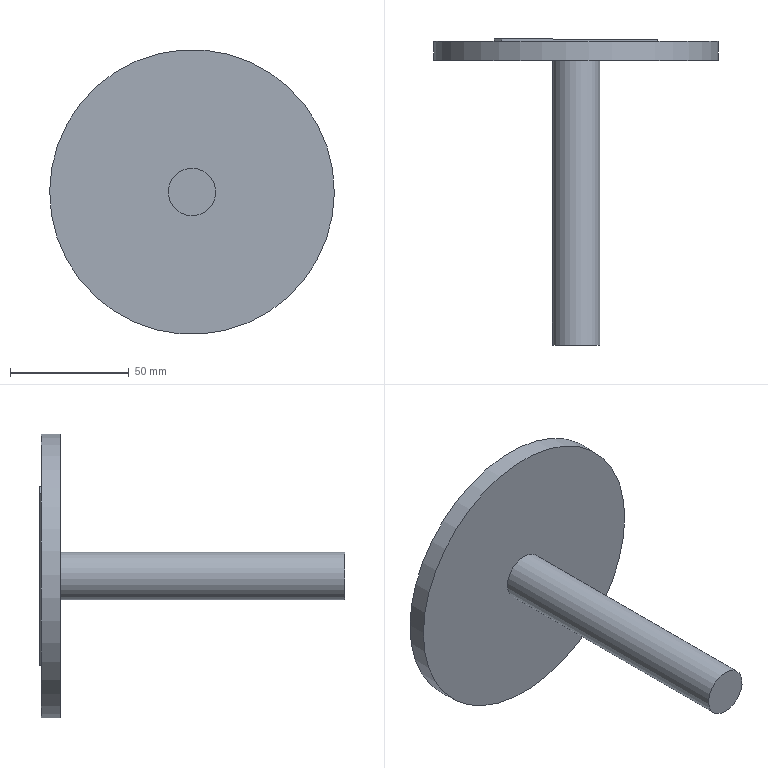Component | NX | MODEL3_3 | 1 solid | 10 faces | box 120 x 129 x 120 mm | volume 128614 mm3 | plane 8 | cylinder 2 | commonest cylinder face diameters 120 x1 20 x1
STEP:
#1=CARTESIAN_POINT('',(0.,0.,0.));
#2=DIRECTION('',(0.,0.,1.));
#3=DIRECTION('',(1.,0.,0.));
#4=AXIS2_PLACEMENT_3D('',#1,#2,#3);
#5=CARTESIAN_POINT('',(-22.229,260.,-82.788));
#6=VERTEX_POINT('',#5);
#7=CARTESIAN_POINT('',(-62.472,260.,-38.286));
#8=DIRECTION('',(0.,-1.,0.));
#9=DIRECTION('',(0.6707,0.,-0.7417));
#10=AXIS2_PLACEMENT_3D('',#7,#8,#9);
#11=CIRCLE('',#10,60.);
#12=CARTESIAN_POINT('',(-62.472,260.,-38.286));
#13=DIRECTION('',(0.,-1.,0.));
#14=DIRECTION('',(-0.7417,0.,-0.6707));
#15=AXIS2_PLACEMENT_3D('',#12,#13,#14);
#16=PLANE('',#15);
#17=CARTESIAN_POINT('',(0.,0.));
#18=DIRECTION('',(0.,1.));
#19=AXIS2_PLACEMENT_2D('',#17,#18);
#20=CIRCLE('',#19,60.);
#21=(GEOMETRIC_REPRESENTATION_CONTEXT(2)PARAMETRIC_REPRESENTATION_CONTEXT()REPRESENTATION_CONTEXT('',''));
#22=DEFINITIONAL_REPRESENTATION('',(#20),#21);
#23=PCURVE('',#16,#22);
#24=CARTESIAN_POINT('',(-62.472,252.,-38.286));
#25=DIRECTION('',(0.,1.,0.));
#26=DIRECTION('',(0.7417,0.,0.6707));
#27=AXIS2_PLACEMENT_3D('',#24,#25,#26);
#28=CYLINDRICAL_SURFACE('',#27,60.);
#29=CARTESIAN_POINT('',(7.854,8.));
#30=DIRECTION('',(-1.,0.));
#31=VECTOR('',#30,1.);
#32=LINE('',#29,#31);
#33=(GEOMETRIC_REPRESENTATION_CONTEXT(2)PARAMETRIC_REPRESENTATION_CONTEXT()REPRESENTATION_CONTEXT('',''));
#34=DEFINITIONAL_REPRESENTATION('',(#32),#33);
#35=PCURVE('',#28,#34);
#36=SURFACE_CURVE('',#11,(#23,#35),.PCURVE_S1.);
#37=EDGE_CURVE('',#6,#6,#36,.T.);
#38=ORIENTED_EDGE('',*,*,#37,.F.);
#39=EDGE_LOOP('',(#38));
#40=FACE_BOUND('',#39,.T.);
#41=CARTESIAN_POINT('',(-96.993,260.,-3.439));
#42=VERTEX_POINT('',#41);
#43=CARTESIAN_POINT('',(-93.683,260.,-0.4456));
#44=VERTEX_POINT('',#43);
#45=CARTESIAN_POINT('',(-96.993,260.,-3.439));
#46=DIRECTION('',(0.7417,0.,0.6707));
#47=VECTOR('',#46,1.);
#48=LINE('',#45,#47);
#49=CARTESIAN_POINT('',(2.231,-49.));
#50=DIRECTION('',(-1.,0.));
#51=VECTOR('',#50,1.);
#52=LINE('',#49,#51);
#53=(GEOMETRIC_REPRESENTATION_CONTEXT(2)PARAMETRIC_REPRESENTATION_CONTEXT()REPRESENTATION_CONTEXT('',''));
#54=DEFINITIONAL_REPRESENTATION('',(#52),#53);
#55=PCURVE('',#16,#54);
#56=CARTESIAN_POINT('',(-96.993,261.,-3.439));
#57=DIRECTION('',(0.6707,0.,-0.7417));
#58=DIRECTION('',(0.7417,0.,0.6707));
#59=AXIS2_PLACEMENT_3D('',#56,#57,#58);
#60=PLANE('',#59);
#61=CARTESIAN_POINT('',(0.,1.));
#62=DIRECTION('',(1.,0.));
#63=VECTOR('',#62,1.);
#64=LINE('',#61,#63);
#65=(GEOMETRIC_REPRESENTATION_CONTEXT(2)PARAMETRIC_REPRESENTATION_CONTEXT()REPRESENTATION_CONTEXT('',''));
#66=DEFINITIONAL_REPRESENTATION('',(#64),#65);
#67=PCURVE('',#60,#66);
#68=SURFACE_CURVE('',#48,(#55,#67),.PCURVE_S1.);
#69=EDGE_CURVE('',#42,#44,#68,.T.);
#70=ORIENTED_EDGE('',*,*,#69,.F.);
#71=CARTESIAN_POINT('',(-31.262,260.,-76.126));
#72=VERTEX_POINT('',#71);
#73=CARTESIAN_POINT('',(-31.262,260.,-76.126));
#74=DIRECTION('',(-0.6707,0.,0.7417));
#75=VECTOR('',#74,1.);
#76=LINE('',#73,#75);
#77=CARTESIAN_POINT('',(2.231,49.));
#78=DIRECTION('',(0.,-1.));
#79=VECTOR('',#78,1.);
#80=LINE('',#77,#79);
#81=(GEOMETRIC_REPRESENTATION_CONTEXT(2)PARAMETRIC_REPRESENTATION_CONTEXT()REPRESENTATION_CONTEXT('',''));
#82=DEFINITIONAL_REPRESENTATION('',(#80),#81);
#83=PCURVE('',#16,#82);
#84=CARTESIAN_POINT('',(-31.262,261.,-76.126));
#85=DIRECTION('',(0.7417,0.,0.6707));
#86=DIRECTION('',(0.,-1.,0.));
#87=AXIS2_PLACEMENT_3D('',#84,#85,#86);
#88=PLANE('',#87);
#89=CARTESIAN_POINT('',(1.,0.));
#90=DIRECTION('',(0.,-1.));
#91=VECTOR('',#90,1.);
#92=LINE('',#89,#91);
#93=(GEOMETRIC_REPRESENTATION_CONTEXT(2)PARAMETRIC_REPRESENTATION_CONTEXT()REPRESENTATION_CONTEXT('',''));
#94=DEFINITIONAL_REPRESENTATION('',(#92),#93);
#95=PCURVE('',#88,#94);
#96=SURFACE_CURVE('',#76,(#83,#95),.PCURVE_S1.);
#97=EDGE_CURVE('',#72,#42,#96,.T.);
#98=ORIENTED_EDGE('',*,*,#97,.F.);
#99=CARTESIAN_POINT('',(-27.952,260.,-73.133));
#100=VERTEX_POINT('',#99);
#101=CARTESIAN_POINT('',(-27.952,260.,-73.133));
#102=DIRECTION('',(-0.7417,0.,-0.6707));
#103=VECTOR('',#102,1.);
#104=LINE('',#101,#103);
#105=CARTESIAN_POINT('',(-2.231,49.));
#106=DIRECTION('',(1.,-0.));
#107=VECTOR('',#106,1.);
#108=LINE('',#105,#107);
#109=(GEOMETRIC_REPRESENTATION_CONTEXT(2)PARAMETRIC_REPRESENTATION_CONTEXT()REPRESENTATION_CONTEXT('',''));
#110=DEFINITIONAL_REPRESENTATION('',(#108),#109);
#111=PCURVE('',#16,#110);
#112=CARTESIAN_POINT('',(-27.952,261.,-73.133));
#113=DIRECTION('',(-0.6707,0.,0.7417));
#114=DIRECTION('',(-0.7417,0.,-0.6707));
#115=AXIS2_PLACEMENT_3D('',#112,#113,#114);
#116=PLANE('',#115);
#117=CARTESIAN_POINT('',(0.,1.));
#118=DIRECTION('',(1.,0.));
#119=VECTOR('',#118,1.);
#120=LINE('',#117,#119);
#121=(GEOMETRIC_REPRESENTATION_CONTEXT(2)PARAMETRIC_REPRESENTATION_CONTEXT()REPRESENTATION_CONTEXT('',''));
#122=DEFINITIONAL_REPRESENTATION('',(#120),#121);
#123=PCURVE('',#116,#122);
#124=SURFACE_CURVE('',#104,(#111,#123),.PCURVE_S1.);
#125=EDGE_CURVE('',#100,#72,#124,.T.);
#126=ORIENTED_EDGE('',*,*,#125,.F.);
#127=CARTESIAN_POINT('',(-93.683,260.,-0.4456));
#128=DIRECTION('',(0.6707,0.,-0.7417));
#129=VECTOR('',#128,1.);
#130=LINE('',#127,#129);
#131=CARTESIAN_POINT('',(-2.231,-49.));
#132=DIRECTION('',(0.,1.));
#133=VECTOR('',#132,1.);
#134=LINE('',#131,#133);
#135=(GEOMETRIC_REPRESENTATION_CONTEXT(2)PARAMETRIC_REPRESENTATION_CONTEXT()REPRESENTATION_CONTEXT('',''));
#136=DEFINITIONAL_REPRESENTATION('',(#134),#135);
#137=PCURVE('',#16,#136);
#138=CARTESIAN_POINT('',(-93.683,261.,-0.4456));
#139=DIRECTION('',(-0.7417,0.,-0.6707));
#140=DIRECTION('',(0.,1.,0.));
#141=AXIS2_PLACEMENT_3D('',#138,#139,#140);
#142=PLANE('',#141);
#143=CARTESIAN_POINT('',(-1.,0.));
#144=DIRECTION('',(0.,1.));
#145=VECTOR('',#144,1.);
#146=LINE('',#143,#145);
#147=(GEOMETRIC_REPRESENTATION_CONTEXT(2)PARAMETRIC_REPRESENTATION_CONTEXT()REPRESENTATION_CONTEXT('',''));
#148=DEFINITIONAL_REPRESENTATION('',(#146),#147);
#149=PCURVE('',#142,#148);
#150=SURFACE_CURVE('',#130,(#137,#149),.PCURVE_S1.);
#151=EDGE_CURVE('',#44,#100,#150,.T.);
#152=ORIENTED_EDGE('',*,*,#151,.F.);
#153=EDGE_LOOP('',(#70,#98,#126,#152));
#154=FACE_BOUND('',#153,.T.);
#155=ADVANCED_FACE('',(#40,#154),#16,.F.);
#156=CARTESIAN_POINT('',(-22.229,252.,-82.788));
#157=VERTEX_POINT('',#156);
#158=CARTESIAN_POINT('',(-62.472,252.,-38.286));
#159=DIRECTION('',(0.,-1.,0.));
#160=DIRECTION('',(0.6707,0.,-0.7417));
#161=AXIS2_PLACEMENT_3D('',#158,#159,#160);
#162=CIRCLE('',#161,60.);
#163=CARTESIAN_POINT('',(7.854,0.));
#164=DIRECTION('',(-1.,0.));
#165=VECTOR('',#164,1.);
#166=LINE('',#163,#165);
#167=(GEOMETRIC_REPRESENTATION_CONTEXT(2)PARAMETRIC_REPRESENTATION_CONTEXT()REPRESENTATION_CONTEXT('',''));
#168=DEFINITIONAL_REPRESENTATION('',(#166),#167);
#169=PCURVE('',#28,#168);
#170=CARTESIAN_POINT('',(-62.472,252.,-38.286));
#171=DIRECTION('',(0.,-1.,0.));
#172=DIRECTION('',(-0.7417,0.,-0.6707));
#173=AXIS2_PLACEMENT_3D('',#170,#171,#172);
#174=PLANE('',#173);
#175=CARTESIAN_POINT('',(0.,0.));
#176=DIRECTION('',(0.,1.));
#177=AXIS2_PLACEMENT_2D('',#175,#176);
#178=CIRCLE('',#177,60.);
#179=(GEOMETRIC_REPRESENTATION_CONTEXT(2)PARAMETRIC_REPRESENTATION_CONTEXT()REPRESENTATION_CONTEXT('',''));
#180=DEFINITIONAL_REPRESENTATION('',(#178),#179);
#181=PCURVE('',#174,#180);
#182=SURFACE_CURVE('',#162,(#169,#181),.PCURVE_S1.);
#183=EDGE_CURVE('',#157,#157,#182,.T.);
#184=ORIENTED_EDGE('',*,*,#183,.F.);
#185=CARTESIAN_POINT('',(-22.229,252.,-82.788));
#186=CARTESIAN_POINT('',(-22.229,260.,-82.788));
#187=B_SPLINE_CURVE_WITH_KNOTS('',1,(#185,#186),.UNSPECIFIED.,.F.,.F.,(2,2),(0.,8.),.PIECEWISE_BEZIER_KNOTS.);
#188=CARTESIAN_POINT('',(7.854,0.));
#189=DIRECTION('',(0.,1.));
#190=VECTOR('',#189,1.);
#191=LINE('',#188,#190);
#192=(GEOMETRIC_REPRESENTATION_CONTEXT(2)PARAMETRIC_REPRESENTATION_CONTEXT()REPRESENTATION_CONTEXT('',''));
#193=DEFINITIONAL_REPRESENTATION('',(#191),#192);
#194=PCURVE('',#28,#193);
#195=CARTESIAN_POINT('',(1.571,0.));
#196=DIRECTION('',(0.,1.));
#197=VECTOR('',#196,1.);
#198=LINE('',#195,#197);
#199=(GEOMETRIC_REPRESENTATION_CONTEXT(2)PARAMETRIC_REPRESENTATION_CONTEXT()REPRESENTATION_CONTEXT('',''));
#200=DEFINITIONAL_REPRESENTATION('',(#198),#199);
#201=PCURVE('',#28,#200);
#202=SEAM_CURVE('',#187,(#194,#201),.PCURVE_S1.);
#203=EDGE_CURVE('',#157,#6,#202,.T.);
#204=ORIENTED_EDGE('',*,*,#203,.T.);
#205=ORIENTED_EDGE('',*,*,#37,.T.);
#206=ORIENTED_EDGE('',*,*,#203,.F.);
#207=EDGE_LOOP('',(#184,#204,#205,#206));
#208=FACE_BOUND('',#207,.T.);
#209=ADVANCED_FACE('',(#208),#28,.T.);
#210=CARTESIAN_POINT('',(-55.765,252.,-45.703));
#211=VERTEX_POINT('',#210);
#212=CARTESIAN_POINT('',(-62.472,252.,-38.286));
#213=DIRECTION('',(0.,-1.,0.));
#214=DIRECTION('',(0.6707,0.,-0.7417));
#215=AXIS2_PLACEMENT_3D('',#212,#213,#214);
#216=CIRCLE('',#215,10.);
#217=CARTESIAN_POINT('',(0.,0.));
#218=DIRECTION('',(-0.,1.));
#219=AXIS2_PLACEMENT_2D('',#217,#218);
#220=CIRCLE('',#219,10.);
#221=(GEOMETRIC_REPRESENTATION_CONTEXT(2)PARAMETRIC_REPRESENTATION_CONTEXT()REPRESENTATION_CONTEXT('',''));
#222=DEFINITIONAL_REPRESENTATION('',(#220),#221);
#223=PCURVE('',#174,#222);
#224=CARTESIAN_POINT('',(-62.472,132.,-38.286));
#225=DIRECTION('',(0.,1.,0.));
#226=DIRECTION('',(0.7417,0.,0.6707));
#227=AXIS2_PLACEMENT_3D('',#224,#225,#226);
#228=CYLINDRICAL_SURFACE('',#227,10.);
#229=CARTESIAN_POINT('',(7.854,120.));
#230=DIRECTION('',(-1.,0.));
#231=VECTOR('',#230,1.);
#232=LINE('',#229,#231);
#233=(GEOMETRIC_REPRESENTATION_CONTEXT(2)PARAMETRIC_REPRESENTATION_CONTEXT()REPRESENTATION_CONTEXT('',''));
#234=DEFINITIONAL_REPRESENTATION('',(#232),#233);
#235=PCURVE('',#228,#234);
#236=SURFACE_CURVE('',#216,(#223,#235),.PCURVE_S1.);
#237=EDGE_CURVE('',#211,#211,#236,.T.);
#238=ORIENTED_EDGE('',*,*,#237,.F.);
#239=EDGE_LOOP('',(#238));
#240=FACE_BOUND('',#239,.T.);
#241=ORIENTED_EDGE('',*,*,#183,.T.);
#242=EDGE_LOOP('',(#241));
#243=FACE_BOUND('',#242,.T.);
#244=ADVANCED_FACE('',(#240,#243),#174,.T.);
#245=CARTESIAN_POINT('',(-55.765,132.,-45.703));
#246=VERTEX_POINT('',#245);
#247=CARTESIAN_POINT('',(-62.472,132.,-38.286));
#248=DIRECTION('',(0.,-1.,0.));
#249=DIRECTION('',(0.6707,0.,-0.7417));
#250=AXIS2_PLACEMENT_3D('',#247,#248,#249);
#251=CIRCLE('',#250,10.);
#252=CARTESIAN_POINT('',(7.854,0.));
#253=DIRECTION('',(-1.,0.));
#254=VECTOR('',#253,1.);
#255=LINE('',#252,#254);
#256=(GEOMETRIC_REPRESENTATION_CONTEXT(2)PARAMETRIC_REPRESENTATION_CONTEXT()REPRESENTATION_CONTEXT('',''));
#257=DEFINITIONAL_REPRESENTATION('',(#255),#256);
#258=PCURVE('',#228,#257);
#259=CARTESIAN_POINT('',(-62.472,132.,-38.286));
#260=DIRECTION('',(0.,-1.,0.));
#261=DIRECTION('',(-0.7417,0.,-0.6707));
#262=AXIS2_PLACEMENT_3D('',#259,#260,#261);
#263=PLANE('',#262);
#264=CARTESIAN_POINT('',(0.,0.));
#265=DIRECTION('',(-0.,1.));
#266=AXIS2_PLACEMENT_2D('',#264,#265);
#267=CIRCLE('',#266,10.);
#268=(GEOMETRIC_REPRESENTATION_CONTEXT(2)PARAMETRIC_REPRESENTATION_CONTEXT()REPRESENTATION_CONTEXT('',''));
#269=DEFINITIONAL_REPRESENTATION('',(#267),#268);
#270=PCURVE('',#263,#269);
#271=SURFACE_CURVE('',#251,(#258,#270),.PCURVE_S1.);
#272=EDGE_CURVE('',#246,#246,#271,.T.);
#273=ORIENTED_EDGE('',*,*,#272,.F.);
#274=CARTESIAN_POINT('',(-55.765,132.,-45.703));
#275=CARTESIAN_POINT('',(-55.765,252.,-45.703));
#276=B_SPLINE_CURVE_WITH_KNOTS('',1,(#274,#275),.UNSPECIFIED.,.F.,.F.,(2,2),(0.,120.),.PIECEWISE_BEZIER_KNOTS.);
#277=CARTESIAN_POINT('',(7.854,0.));
#278=DIRECTION('',(0.,1.));
#279=VECTOR('',#278,1.);
#280=LINE('',#277,#279);
#281=(GEOMETRIC_REPRESENTATION_CONTEXT(2)PARAMETRIC_REPRESENTATION_CONTEXT()REPRESENTATION_CONTEXT('',''));
#282=DEFINITIONAL_REPRESENTATION('',(#280),#281);
#283=PCURVE('',#228,#282);
#284=CARTESIAN_POINT('',(1.571,0.));
#285=DIRECTION('',(0.,1.));
#286=VECTOR('',#285,1.);
#287=LINE('',#284,#286);
#288=(GEOMETRIC_REPRESENTATION_CONTEXT(2)PARAMETRIC_REPRESENTATION_CONTEXT()REPRESENTATION_CONTEXT('',''));
#289=DEFINITIONAL_REPRESENTATION('',(#287),#288);
#290=PCURVE('',#228,#289);
#291=SEAM_CURVE('',#276,(#283,#290),.PCURVE_S1.);
#292=EDGE_CURVE('',#246,#211,#291,.T.);
#293=ORIENTED_EDGE('',*,*,#292,.T.);
#294=ORIENTED_EDGE('',*,*,#237,.T.);
#295=ORIENTED_EDGE('',*,*,#292,.F.);
#296=EDGE_LOOP('',(#273,#293,#294,#295));
#297=FACE_BOUND('',#296,.T.);
#298=ADVANCED_FACE('',(#297),#228,.T.);
#299=ORIENTED_EDGE('',*,*,#272,.T.);
#300=EDGE_LOOP('',(#299));
#301=FACE_BOUND('',#300,.T.);
#302=ADVANCED_FACE('',(#301),#263,.T.);
#303=ORIENTED_EDGE('',*,*,#69,.T.);
#304=CARTESIAN_POINT('',(-93.683,261.,-0.4456));
#305=VERTEX_POINT('',#304);
#306=CARTESIAN_POINT('',(-93.683,261.,-0.4456));
#307=DIRECTION('',(0.,-1.,0.));
#308=VECTOR('',#307,1.);
#309=LINE('',#306,#308);
#310=CARTESIAN_POINT('',(4.462,0.));
#311=DIRECTION('',(0.,1.));
#312=VECTOR('',#311,1.);
#313=LINE('',#310,#312);
#314=(GEOMETRIC_REPRESENTATION_CONTEXT(2)PARAMETRIC_REPRESENTATION_CONTEXT()REPRESENTATION_CONTEXT('',''));
#315=DEFINITIONAL_REPRESENTATION('',(#313),#314);
#316=PCURVE('',#60,#315);
#317=CARTESIAN_POINT('',(0.,0.));
#318=DIRECTION('',(-1.,0.));
#319=VECTOR('',#318,1.);
#320=LINE('',#317,#319);
#321=(GEOMETRIC_REPRESENTATION_CONTEXT(2)PARAMETRIC_REPRESENTATION_CONTEXT()REPRESENTATION_CONTEXT('',''));
#322=DEFINITIONAL_REPRESENTATION('',(#320),#321);
#323=PCURVE('',#142,#322);
#324=SURFACE_CURVE('',#309,(#316,#323),.PCURVE_S1.);
#325=EDGE_CURVE('',#305,#44,#324,.T.);
#326=ORIENTED_EDGE('',*,*,#325,.F.);
#327=CARTESIAN_POINT('',(-96.993,261.,-3.439));
#328=VERTEX_POINT('',#327);
#329=CARTESIAN_POINT('',(-96.993,261.,-3.439));
#330=DIRECTION('',(0.7417,0.,0.6707));
#331=VECTOR('',#330,1.);
#332=LINE('',#329,#331);
#333=CARTESIAN_POINT('',(0.,0.));
#334=DIRECTION('',(1.,0.));
#335=VECTOR('',#334,1.);
#336=LINE('',#333,#335);
#337=(GEOMETRIC_REPRESENTATION_CONTEXT(2)PARAMETRIC_REPRESENTATION_CONTEXT()REPRESENTATION_CONTEXT('',''));
#338=DEFINITIONAL_REPRESENTATION('',(#336),#337);
#339=PCURVE('',#60,#338);
#340=CARTESIAN_POINT('',(-62.472,261.,-38.286));
#341=DIRECTION('',(0.,1.,0.));
#342=DIRECTION('',(0.7417,0.,0.6707));
#343=AXIS2_PLACEMENT_3D('',#340,#341,#342);
#344=PLANE('',#343);
#345=CARTESIAN_POINT('',(-2.231,-49.));
#346=DIRECTION('',(1.,0.));
#347=VECTOR('',#346,1.);
#348=LINE('',#345,#347);
#349=(GEOMETRIC_REPRESENTATION_CONTEXT(2)PARAMETRIC_REPRESENTATION_CONTEXT()REPRESENTATION_CONTEXT('',''));
#350=DEFINITIONAL_REPRESENTATION('',(#348),#349);
#351=PCURVE('',#344,#350);
#352=SURFACE_CURVE('',#332,(#339,#351),.PCURVE_S1.);
#353=EDGE_CURVE('',#328,#305,#352,.T.);
#354=ORIENTED_EDGE('',*,*,#353,.F.);
#355=CARTESIAN_POINT('',(-96.993,261.,-3.439));
#356=DIRECTION('',(0.,-1.,0.));
#357=VECTOR('',#356,1.);
#358=LINE('',#355,#357);
#359=CARTESIAN_POINT('',(0.,0.));
#360=DIRECTION('',(0.,1.));
#361=VECTOR('',#360,1.);
#362=LINE('',#359,#361);
#363=(GEOMETRIC_REPRESENTATION_CONTEXT(2)PARAMETRIC_REPRESENTATION_CONTEXT()REPRESENTATION_CONTEXT('',''));
#364=DEFINITIONAL_REPRESENTATION('',(#362),#363);
#365=PCURVE('',#60,#364);
#366=CARTESIAN_POINT('',(0.,-98.));
#367=DIRECTION('',(1.,0.));
#368=VECTOR('',#367,1.);
#369=LINE('',#366,#368);
#370=(GEOMETRIC_REPRESENTATION_CONTEXT(2)PARAMETRIC_REPRESENTATION_CONTEXT()REPRESENTATION_CONTEXT('',''));
#371=DEFINITIONAL_REPRESENTATION('',(#369),#370);
#372=PCURVE('',#88,#371);
#373=SURFACE_CURVE('',#358,(#365,#372),.PCURVE_S1.);
#374=EDGE_CURVE('',#328,#42,#373,.T.);
#375=ORIENTED_EDGE('',*,*,#374,.T.);
#376=EDGE_LOOP('',(#303,#326,#354,#375));
#377=FACE_BOUND('',#376,.T.);
#378=ADVANCED_FACE('',(#377),#60,.F.);
#379=ORIENTED_EDGE('',*,*,#151,.T.);
#380=CARTESIAN_POINT('',(-27.952,261.,-73.133));
#381=VERTEX_POINT('',#380);
#382=CARTESIAN_POINT('',(-27.952,261.,-73.133));
#383=DIRECTION('',(0.,-1.,0.));
#384=VECTOR('',#383,1.);
#385=LINE('',#382,#384);
#386=CARTESIAN_POINT('',(0.,98.));
#387=DIRECTION('',(-1.,0.));
#388=VECTOR('',#387,1.);
#389=LINE('',#386,#388);
#390=(GEOMETRIC_REPRESENTATION_CONTEXT(2)PARAMETRIC_REPRESENTATION_CONTEXT()REPRESENTATION_CONTEXT('',''));
#391=DEFINITIONAL_REPRESENTATION('',(#389),#390);
#392=PCURVE('',#142,#391);
#393=CARTESIAN_POINT('',(0.,0.));
#394=DIRECTION('',(0.,1.));
#395=VECTOR('',#394,1.);
#396=LINE('',#393,#395);
#397=(GEOMETRIC_REPRESENTATION_CONTEXT(2)PARAMETRIC_REPRESENTATION_CONTEXT()REPRESENTATION_CONTEXT('',''));
#398=DEFINITIONAL_REPRESENTATION('',(#396),#397);
#399=PCURVE('',#116,#398);
#400=SURFACE_CURVE('',#385,(#392,#399),.PCURVE_S1.);
#401=EDGE_CURVE('',#381,#100,#400,.T.);
#402=ORIENTED_EDGE('',*,*,#401,.F.);
#403=CARTESIAN_POINT('',(-93.683,261.,-0.4456));
#404=DIRECTION('',(0.6707,0.,-0.7417));
#405=VECTOR('',#404,1.);
#406=LINE('',#403,#405);
#407=CARTESIAN_POINT('',(0.,0.));
#408=DIRECTION('',(0.,1.));
#409=VECTOR('',#408,1.);
#410=LINE('',#407,#409);
#411=(GEOMETRIC_REPRESENTATION_CONTEXT(2)PARAMETRIC_REPRESENTATION_CONTEXT()REPRESENTATION_CONTEXT('',''));
#412=DEFINITIONAL_REPRESENTATION('',(#410),#411);
#413=PCURVE('',#142,#412);
#414=CARTESIAN_POINT('',(2.231,-49.));
#415=DIRECTION('',(0.,1.));
#416=VECTOR('',#415,1.);
#417=LINE('',#414,#416);
#418=(GEOMETRIC_REPRESENTATION_CONTEXT(2)PARAMETRIC_REPRESENTATION_CONTEXT()REPRESENTATION_CONTEXT('',''));
#419=DEFINITIONAL_REPRESENTATION('',(#417),#418);
#420=PCURVE('',#344,#419);
#421=SURFACE_CURVE('',#406,(#413,#420),.PCURVE_S1.);
#422=EDGE_CURVE('',#305,#381,#421,.T.);
#423=ORIENTED_EDGE('',*,*,#422,.F.);
#424=ORIENTED_EDGE('',*,*,#325,.T.);
#425=EDGE_LOOP('',(#379,#402,#423,#424));
#426=FACE_BOUND('',#425,.T.);
#427=ADVANCED_FACE('',(#426),#142,.F.);
#428=ORIENTED_EDGE('',*,*,#125,.T.);
#429=CARTESIAN_POINT('',(-31.262,261.,-76.126));
#430=VERTEX_POINT('',#429);
#431=CARTESIAN_POINT('',(-31.262,261.,-76.126));
#432=DIRECTION('',(0.,-1.,0.));
#433=VECTOR('',#432,1.);
#434=LINE('',#431,#433);
#435=CARTESIAN_POINT('',(4.462,0.));
#436=DIRECTION('',(0.,1.));
#437=VECTOR('',#436,1.);
#438=LINE('',#435,#437);
#439=(GEOMETRIC_REPRESENTATION_CONTEXT(2)PARAMETRIC_REPRESENTATION_CONTEXT()REPRESENTATION_CONTEXT('',''));
#440=DEFINITIONAL_REPRESENTATION('',(#438),#439);
#441=PCURVE('',#116,#440);
#442=CARTESIAN_POINT('',(0.,0.));
#443=DIRECTION('',(1.,0.));
#444=VECTOR('',#443,1.);
#445=LINE('',#442,#444);
#446=(GEOMETRIC_REPRESENTATION_CONTEXT(2)PARAMETRIC_REPRESENTATION_CONTEXT()REPRESENTATION_CONTEXT('',''));
#447=DEFINITIONAL_REPRESENTATION('',(#445),#446);
#448=PCURVE('',#88,#447);
#449=SURFACE_CURVE('',#434,(#441,#448),.PCURVE_S1.);
#450=EDGE_CURVE('',#430,#72,#449,.T.);
#451=ORIENTED_EDGE('',*,*,#450,.F.);
#452=CARTESIAN_POINT('',(-27.952,261.,-73.133));
#453=DIRECTION('',(-0.7417,0.,-0.6707));
#454=VECTOR('',#453,1.);
#455=LINE('',#452,#454);
#456=CARTESIAN_POINT('',(0.,0.));
#457=DIRECTION('',(1.,0.));
#458=VECTOR('',#457,1.);
#459=LINE('',#456,#458);
#460=(GEOMETRIC_REPRESENTATION_CONTEXT(2)PARAMETRIC_REPRESENTATION_CONTEXT()REPRESENTATION_CONTEXT('',''));
#461=DEFINITIONAL_REPRESENTATION('',(#459),#460);
#462=PCURVE('',#116,#461);
#463=CARTESIAN_POINT('',(2.231,49.));
#464=DIRECTION('',(-1.,-0.));
#465=VECTOR('',#464,1.);
#466=LINE('',#463,#465);
#467=(GEOMETRIC_REPRESENTATION_CONTEXT(2)PARAMETRIC_REPRESENTATION_CONTEXT()REPRESENTATION_CONTEXT('',''));
#468=DEFINITIONAL_REPRESENTATION('',(#466),#467);
#469=PCURVE('',#344,#468);
#470=SURFACE_CURVE('',#455,(#462,#469),.PCURVE_S1.);
#471=EDGE_CURVE('',#381,#430,#470,.T.);
#472=ORIENTED_EDGE('',*,*,#471,.F.);
#473=ORIENTED_EDGE('',*,*,#401,.T.);
#474=EDGE_LOOP('',(#428,#451,#472,#473));
#475=FACE_BOUND('',#474,.T.);
#476=ADVANCED_FACE('',(#475),#116,.F.);
#477=ORIENTED_EDGE('',*,*,#97,.T.);
#478=ORIENTED_EDGE('',*,*,#374,.F.);
#479=CARTESIAN_POINT('',(-31.262,261.,-76.126));
#480=DIRECTION('',(-0.6707,0.,0.7417));
#481=VECTOR('',#480,1.);
#482=LINE('',#479,#481);
#483=CARTESIAN_POINT('',(0.,0.));
#484=DIRECTION('',(0.,-1.));
#485=VECTOR('',#484,1.);
#486=LINE('',#483,#485);
#487=(GEOMETRIC_REPRESENTATION_CONTEXT(2)PARAMETRIC_REPRESENTATION_CONTEXT()REPRESENTATION_CONTEXT('',''));
#488=DEFINITIONAL_REPRESENTATION('',(#486),#487);
#489=PCURVE('',#88,#488);
#490=CARTESIAN_POINT('',(-2.231,49.));
#491=DIRECTION('',(0.,-1.));
#492=VECTOR('',#491,1.);
#493=LINE('',#490,#492);
#494=(GEOMETRIC_REPRESENTATION_CONTEXT(2)PARAMETRIC_REPRESENTATION_CONTEXT()REPRESENTATION_CONTEXT('',''));
#495=DEFINITIONAL_REPRESENTATION('',(#493),#494);
#496=PCURVE('',#344,#495);
#497=SURFACE_CURVE('',#482,(#489,#496),.PCURVE_S1.);
#498=EDGE_CURVE('',#430,#328,#497,.T.);
#499=ORIENTED_EDGE('',*,*,#498,.F.);
#500=ORIENTED_EDGE('',*,*,#450,.T.);
#501=EDGE_LOOP('',(#477,#478,#499,#500));
#502=FACE_BOUND('',#501,.T.);
#503=ADVANCED_FACE('',(#502),#88,.F.);
#504=ORIENTED_EDGE('',*,*,#353,.T.);
#505=ORIENTED_EDGE('',*,*,#422,.T.);
#506=ORIENTED_EDGE('',*,*,#471,.T.);
#507=ORIENTED_EDGE('',*,*,#498,.T.);
#508=EDGE_LOOP('',(#504,#505,#506,#507));
#509=FACE_BOUND('',#508,.T.);
#510=ADVANCED_FACE('',(#509),#344,.T.);
#511=CLOSED_SHELL('',(#155,#209,#244,#298,#302,#378,#427,#476,#503,#510));
#512=MANIFOLD_SOLID_BREP('',#511);
#513=(LENGTH_UNIT()NAMED_UNIT(*)SI_UNIT(.MILLI.,.METRE.));
#514=UNCERTAINTY_MEASURE_WITH_UNIT(LENGTH_MEASURE(0.000002),#513,'','');
#515=(NAMED_UNIT(*)PLANE_ANGLE_UNIT()SI_UNIT($,.RADIAN.));
#516=(NAMED_UNIT(*)SI_UNIT($,.STERADIAN.)SOLID_ANGLE_UNIT());
#517=(GEOMETRIC_REPRESENTATION_CONTEXT(3)GLOBAL_UNCERTAINTY_ASSIGNED_CONTEXT((#514))GLOBAL_UNIT_ASSIGNED_CONTEXT((#513,#515,#516))REPRESENTATION_CONTEXT('',''));
#518=ADVANCED_BREP_SHAPE_REPRESENTATION('',(#4,#512),#517);